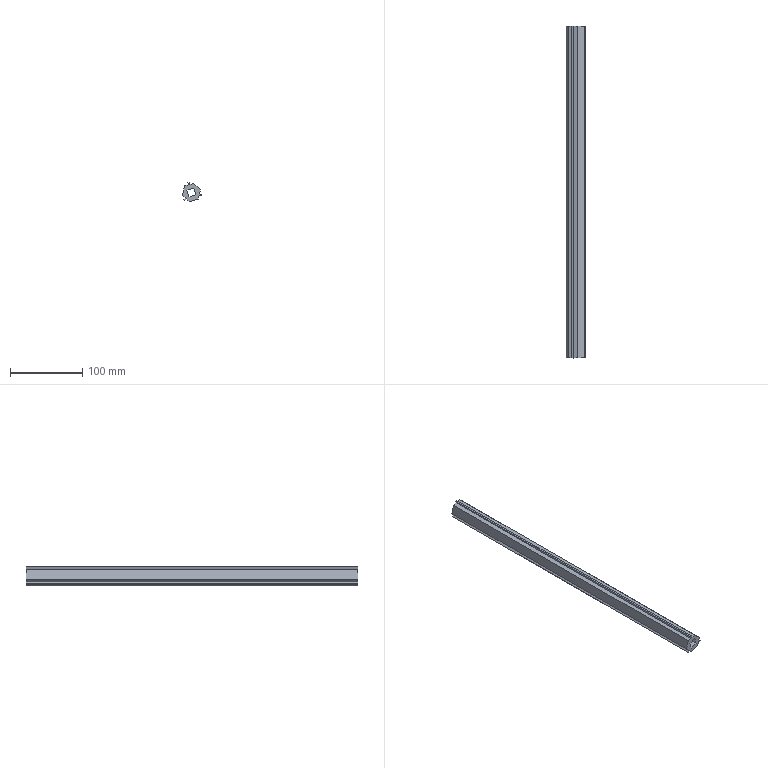Component | SolidWorks | Drive-1 | 1 solid | 24 faces | box 26.58 x 460 x 26.59 mm | volume 164254 mm3 | plane 24
STEP:
#1=CARTESIAN_POINT('',(-2.72,0.992,35.851));
#2=VERTEX_POINT('',#1);
#3=CARTESIAN_POINT('',(-2.928,0.992,35.792));
#4=VERTEX_POINT('',#3);
#5=CARTESIAN_POINT('',(-2.72,0.992,35.851));
#6=DIRECTION('',(-0.962,-0.,-0.273));
#7=VECTOR('',#6,39.37);
#8=LINE('',#5,#7);
#9=EDGE_CURVE('',#2,#4,#8,.T.);
#10=ORIENTED_EDGE('',*,*,#9,.T.);
#11=CARTESIAN_POINT('',(-3.053,0.992,35.296));
#12=VERTEX_POINT('',#11);
#13=CARTESIAN_POINT('',(-2.928,0.992,35.792));
#14=DIRECTION('',(-0.2446,0.,-0.9696));
#15=VECTOR('',#14,39.37);
#16=LINE('',#13,#15);
#17=EDGE_CURVE('',#4,#12,#16,.T.);
#18=ORIENTED_EDGE('',*,*,#17,.T.);
#19=CARTESIAN_POINT('',(-2.898,0.992,35.145));
#20=VERTEX_POINT('',#19);
#21=CARTESIAN_POINT('',(-3.053,0.992,35.296));
#22=DIRECTION('',(0.7175,0.,-0.6966));
#23=VECTOR('',#22,39.37);
#24=LINE('',#21,#23);
#25=EDGE_CURVE('',#12,#20,#24,.T.);
#26=ORIENTED_EDGE('',*,*,#25,.T.);
#27=CARTESIAN_POINT('',(-2.98,0.992,35.06));
#28=VERTEX_POINT('',#27);
#29=CARTESIAN_POINT('',(-2.898,0.992,35.145));
#30=DIRECTION('',(-0.6966,0.,-0.7175));
#31=VECTOR('',#30,39.37);
#32=LINE('',#29,#31);
#33=EDGE_CURVE('',#20,#28,#32,.T.);
#34=ORIENTED_EDGE('',*,*,#33,.T.);
#35=CARTESIAN_POINT('',(-2.924,0.992,35.005));
#36=VERTEX_POINT('',#35);
#37=CARTESIAN_POINT('',(-2.98,0.992,35.06));
#38=DIRECTION('',(0.7175,0.,-0.6966));
#39=VECTOR('',#38,39.37);
#40=LINE('',#37,#39);
#41=EDGE_CURVE('',#28,#36,#40,.T.);
#42=ORIENTED_EDGE('',*,*,#41,.T.);
#43=CARTESIAN_POINT('',(-2.841,0.992,35.09));
#44=VERTEX_POINT('',#43);
#45=CARTESIAN_POINT('',(-2.924,0.992,35.005));
#46=DIRECTION('',(0.6966,-0.,0.7175));
#47=VECTOR('',#46,39.37);
#48=LINE('',#45,#47);
#49=EDGE_CURVE('',#36,#44,#48,.T.);
#50=ORIENTED_EDGE('',*,*,#49,.T.);
#51=CARTESIAN_POINT('',(-2.686,0.992,34.939));
#52=VERTEX_POINT('',#51);
#53=CARTESIAN_POINT('',(-2.841,0.992,35.09));
#54=DIRECTION('',(0.7175,0.,-0.6966));
#55=VECTOR('',#54,39.37);
#56=LINE('',#53,#55);
#57=EDGE_CURVE('',#44,#52,#56,.T.);
#58=ORIENTED_EDGE('',*,*,#57,.T.);
#59=CARTESIAN_POINT('',(-2.194,0.992,35.079));
#60=VERTEX_POINT('',#59);
#61=CARTESIAN_POINT('',(-2.686,0.992,34.939));
#62=DIRECTION('',(0.962,0.,0.273));
#63=VECTOR('',#62,39.37);
#64=LINE('',#61,#63);
#65=EDGE_CURVE('',#52,#60,#64,.T.);
#66=ORIENTED_EDGE('',*,*,#65,.T.);
#67=CARTESIAN_POINT('',(-2.141,0.992,35.289));
#68=VERTEX_POINT('',#67);
#69=CARTESIAN_POINT('',(-2.194,0.992,35.079));
#70=DIRECTION('',(0.2446,-0.,0.9696));
#71=VECTOR('',#70,39.37);
#72=LINE('',#69,#71);
#73=EDGE_CURVE('',#60,#68,#72,.T.);
#74=ORIENTED_EDGE('',*,*,#73,.T.);
#75=CARTESIAN_POINT('',(-2.026,0.992,35.26));
#76=VERTEX_POINT('',#75);
#77=CARTESIAN_POINT('',(-2.026,0.992,35.26));
#78=DIRECTION('',(0.9696,0.,-0.2446));
#79=VECTOR('',#78,39.37);
#80=LINE('',#77,#79);
#81=EDGE_CURVE('',#68,#76,#80,.T.);
#82=ORIENTED_EDGE('',*,*,#81,.T.);
#83=CARTESIAN_POINT('',(-2.007,0.992,35.336));
#84=VERTEX_POINT('',#83);
#85=CARTESIAN_POINT('',(-2.007,0.992,35.336));
#86=DIRECTION('',(0.2446,-0.,0.9696));
#87=VECTOR('',#86,39.37);
#88=LINE('',#85,#87);
#89=EDGE_CURVE('',#76,#84,#88,.T.);
#90=ORIENTED_EDGE('',*,*,#89,.T.);
#91=CARTESIAN_POINT('',(-2.121,0.992,35.365));
#92=VERTEX_POINT('',#91);
#93=CARTESIAN_POINT('',(-2.121,0.992,35.365));
#94=DIRECTION('',(-0.9696,-0.,0.2446));
#95=VECTOR('',#94,39.37);
#96=LINE('',#93,#95);
#97=EDGE_CURVE('',#84,#92,#96,.T.);
#98=ORIENTED_EDGE('',*,*,#97,.T.);
#99=CARTESIAN_POINT('',(-2.068,0.992,35.575));
#100=VERTEX_POINT('',#99);
#101=CARTESIAN_POINT('',(-2.121,0.992,35.365));
#102=DIRECTION('',(0.2446,-0.,0.9696));
#103=VECTOR('',#102,39.37);
#104=LINE('',#101,#103);
#105=EDGE_CURVE('',#92,#100,#104,.T.);
#106=ORIENTED_EDGE('',*,*,#105,.T.);
#107=CARTESIAN_POINT('',(-2.436,0.992,35.932));
#108=VERTEX_POINT('',#107);
#109=CARTESIAN_POINT('',(-2.068,0.992,35.575));
#110=DIRECTION('',(-0.7175,-0.,0.6966));
#111=VECTOR('',#110,39.37);
#112=LINE('',#109,#111);
#113=EDGE_CURVE('',#100,#108,#112,.T.);
#114=ORIENTED_EDGE('',*,*,#113,.T.);
#115=CARTESIAN_POINT('',(-2.644,0.992,35.873));
#116=VERTEX_POINT('',#115);
#117=CARTESIAN_POINT('',(-2.436,0.992,35.932));
#118=DIRECTION('',(-0.962,-0.,-0.273));
#119=VECTOR('',#118,39.37);
#120=LINE('',#117,#119);
#121=EDGE_CURVE('',#108,#116,#120,.T.);
#122=ORIENTED_EDGE('',*,*,#121,.T.);
#123=CARTESIAN_POINT('',(-2.676,0.992,35.986));
#124=VERTEX_POINT('',#123);
#125=CARTESIAN_POINT('',(-2.676,0.992,35.986));
#126=DIRECTION('',(-0.273,-0.,0.962));
#127=VECTOR('',#126,39.37);
#128=LINE('',#125,#127);
#129=EDGE_CURVE('',#116,#124,#128,.T.);
#130=ORIENTED_EDGE('',*,*,#129,.T.);
#131=CARTESIAN_POINT('',(-2.752,0.992,35.965));
#132=VERTEX_POINT('',#131);
#133=CARTESIAN_POINT('',(-2.752,0.992,35.965));
#134=DIRECTION('',(-0.962,-0.,-0.273));
#135=VECTOR('',#134,39.37);
#136=LINE('',#133,#135);
#137=EDGE_CURVE('',#124,#132,#136,.T.);
#138=ORIENTED_EDGE('',*,*,#137,.T.);
#139=CARTESIAN_POINT('',(-2.72,0.992,35.851));
#140=DIRECTION('',(0.273,0.,-0.962));
#141=VECTOR('',#140,39.37);
#142=LINE('',#139,#141);
#143=EDGE_CURVE('',#132,#2,#142,.T.);
#144=ORIENTED_EDGE('',*,*,#143,.T.);
#145=EDGE_LOOP('',(#10,#18,#26,#34,#42,#50,#58,#66,#74,#82,#90,#98,#106,#114,#122,#130,#138,#144));
#146=FACE_OUTER_BOUND('',#145,.T.);
#147=CARTESIAN_POINT('',(-2.425,0.992,35.679));
#148=VERTEX_POINT('',#147);
#149=CARTESIAN_POINT('',(-2.804,0.992,35.571));
#150=VERTEX_POINT('',#149);
#151=CARTESIAN_POINT('',(-2.804,0.992,35.571));
#152=DIRECTION('',(-0.962,-0.,-0.273));
#153=VECTOR('',#152,39.37);
#154=LINE('',#151,#153);
#155=EDGE_CURVE('',#148,#150,#154,.T.);
#156=ORIENTED_EDGE('',*,*,#155,.F.);
#157=CARTESIAN_POINT('',(-2.318,0.992,35.3));
#158=VERTEX_POINT('',#157);
#159=CARTESIAN_POINT('',(-2.425,0.992,35.679));
#160=DIRECTION('',(-0.273,-0.,0.962));
#161=VECTOR('',#160,39.37);
#162=LINE('',#159,#161);
#163=EDGE_CURVE('',#158,#148,#162,.T.);
#164=ORIENTED_EDGE('',*,*,#163,.F.);
#165=CARTESIAN_POINT('',(-2.696,0.992,35.192));
#166=VERTEX_POINT('',#165);
#167=CARTESIAN_POINT('',(-2.696,0.992,35.192));
#168=DIRECTION('',(0.962,0.,0.273));
#169=VECTOR('',#168,39.37);
#170=LINE('',#167,#169);
#171=EDGE_CURVE('',#166,#158,#170,.T.);
#172=ORIENTED_EDGE('',*,*,#171,.F.);
#173=CARTESIAN_POINT('',(-2.804,0.992,35.571));
#174=DIRECTION('',(0.273,0.,-0.962));
#175=VECTOR('',#174,39.37);
#176=LINE('',#173,#175);
#177=EDGE_CURVE('',#150,#166,#176,.T.);
#178=ORIENTED_EDGE('',*,*,#177,.F.);
#179=EDGE_LOOP('',(#156,#164,#172,#178));
#180=FACE_BOUND('',#179,.T.);
#181=CARTESIAN_POINT('',(-2.561,0.992,35.436));
#182=DIRECTION('',(0.,-1.,-0.));
#183=DIRECTION('',(0.962,0.,0.273));
#184=AXIS2_PLACEMENT_3D('',#181,#182,#183);
#185=PLANE('',#184);
#186=ADVANCED_FACE('',(#146,#180),#185,.T.);
#187=CARTESIAN_POINT('',(-2.72,19.102,35.851));
#188=VERTEX_POINT('',#187);
#189=CARTESIAN_POINT('',(-2.928,19.102,35.792));
#190=VERTEX_POINT('',#189);
#191=CARTESIAN_POINT('',(-2.72,19.102,35.851));
#192=DIRECTION('',(-0.962,-0.,-0.273));
#193=VECTOR('',#192,39.37);
#194=LINE('',#191,#193);
#195=EDGE_CURVE('',#188,#190,#194,.T.);
#196=ORIENTED_EDGE('',*,*,#195,.F.);
#197=CARTESIAN_POINT('',(-2.752,19.102,35.965));
#198=VERTEX_POINT('',#197);
#199=CARTESIAN_POINT('',(-2.72,19.102,35.851));
#200=DIRECTION('',(0.273,0.,-0.962));
#201=VECTOR('',#200,39.37);
#202=LINE('',#199,#201);
#203=EDGE_CURVE('',#198,#188,#202,.T.);
#204=ORIENTED_EDGE('',*,*,#203,.F.);
#205=CARTESIAN_POINT('',(-2.676,19.102,35.986));
#206=VERTEX_POINT('',#205);
#207=CARTESIAN_POINT('',(-2.752,19.102,35.965));
#208=DIRECTION('',(-0.962,-0.,-0.273));
#209=VECTOR('',#208,39.37);
#210=LINE('',#207,#209);
#211=EDGE_CURVE('',#206,#198,#210,.T.);
#212=ORIENTED_EDGE('',*,*,#211,.F.);
#213=CARTESIAN_POINT('',(-2.644,19.102,35.873));
#214=VERTEX_POINT('',#213);
#215=CARTESIAN_POINT('',(-2.676,19.102,35.986));
#216=DIRECTION('',(-0.273,-0.,0.962));
#217=VECTOR('',#216,39.37);
#218=LINE('',#215,#217);
#219=EDGE_CURVE('',#214,#206,#218,.T.);
#220=ORIENTED_EDGE('',*,*,#219,.F.);
#221=CARTESIAN_POINT('',(-2.436,19.102,35.932));
#222=VERTEX_POINT('',#221);
#223=CARTESIAN_POINT('',(-2.436,19.102,35.932));
#224=DIRECTION('',(-0.962,-0.,-0.273));
#225=VECTOR('',#224,39.37);
#226=LINE('',#223,#225);
#227=EDGE_CURVE('',#222,#214,#226,.T.);
#228=ORIENTED_EDGE('',*,*,#227,.F.);
#229=CARTESIAN_POINT('',(-2.068,19.102,35.575));
#230=VERTEX_POINT('',#229);
#231=CARTESIAN_POINT('',(-2.068,19.102,35.575));
#232=DIRECTION('',(-0.7175,-0.,0.6966));
#233=VECTOR('',#232,39.37);
#234=LINE('',#231,#233);
#235=EDGE_CURVE('',#230,#222,#234,.T.);
#236=ORIENTED_EDGE('',*,*,#235,.F.);
#237=CARTESIAN_POINT('',(-2.121,19.102,35.365));
#238=VERTEX_POINT('',#237);
#239=CARTESIAN_POINT('',(-2.121,19.102,35.365));
#240=DIRECTION('',(0.2446,-0.,0.9696));
#241=VECTOR('',#240,39.37);
#242=LINE('',#239,#241);
#243=EDGE_CURVE('',#238,#230,#242,.T.);
#244=ORIENTED_EDGE('',*,*,#243,.F.);
#245=CARTESIAN_POINT('',(-2.007,19.102,35.336));
#246=VERTEX_POINT('',#245);
#247=CARTESIAN_POINT('',(-2.121,19.102,35.365));
#248=DIRECTION('',(-0.9696,-0.,0.2446));
#249=VECTOR('',#248,39.37);
#250=LINE('',#247,#249);
#251=EDGE_CURVE('',#246,#238,#250,.T.);
#252=ORIENTED_EDGE('',*,*,#251,.F.);
#253=CARTESIAN_POINT('',(-2.026,19.102,35.26));
#254=VERTEX_POINT('',#253);
#255=CARTESIAN_POINT('',(-2.007,19.102,35.336));
#256=DIRECTION('',(0.2446,-0.,0.9696));
#257=VECTOR('',#256,39.37);
#258=LINE('',#255,#257);
#259=EDGE_CURVE('',#254,#246,#258,.T.);
#260=ORIENTED_EDGE('',*,*,#259,.F.);
#261=CARTESIAN_POINT('',(-2.141,19.102,35.289));
#262=VERTEX_POINT('',#261);
#263=CARTESIAN_POINT('',(-2.026,19.102,35.26));
#264=DIRECTION('',(0.9696,0.,-0.2446));
#265=VECTOR('',#264,39.37);
#266=LINE('',#263,#265);
#267=EDGE_CURVE('',#262,#254,#266,.T.);
#268=ORIENTED_EDGE('',*,*,#267,.F.);
#269=CARTESIAN_POINT('',(-2.194,19.102,35.079));
#270=VERTEX_POINT('',#269);
#271=CARTESIAN_POINT('',(-2.194,19.102,35.079));
#272=DIRECTION('',(0.2446,-0.,0.9696));
#273=VECTOR('',#272,39.37);
#274=LINE('',#271,#273);
#275=EDGE_CURVE('',#270,#262,#274,.T.);
#276=ORIENTED_EDGE('',*,*,#275,.F.);
#277=CARTESIAN_POINT('',(-2.686,19.102,34.939));
#278=VERTEX_POINT('',#277);
#279=CARTESIAN_POINT('',(-2.686,19.102,34.939));
#280=DIRECTION('',(0.962,0.,0.273));
#281=VECTOR('',#280,39.37);
#282=LINE('',#279,#281);
#283=EDGE_CURVE('',#278,#270,#282,.T.);
#284=ORIENTED_EDGE('',*,*,#283,.F.);
#285=CARTESIAN_POINT('',(-2.841,19.102,35.09));
#286=VERTEX_POINT('',#285);
#287=CARTESIAN_POINT('',(-2.841,19.102,35.09));
#288=DIRECTION('',(0.7175,0.,-0.6966));
#289=VECTOR('',#288,39.37);
#290=LINE('',#287,#289);
#291=EDGE_CURVE('',#286,#278,#290,.T.);
#292=ORIENTED_EDGE('',*,*,#291,.F.);
#293=CARTESIAN_POINT('',(-2.924,19.102,35.005));
#294=VERTEX_POINT('',#293);
#295=CARTESIAN_POINT('',(-2.924,19.102,35.005));
#296=DIRECTION('',(0.6966,-0.,0.7175));
#297=VECTOR('',#296,39.37);
#298=LINE('',#295,#297);
#299=EDGE_CURVE('',#294,#286,#298,.T.);
#300=ORIENTED_EDGE('',*,*,#299,.F.);
#301=CARTESIAN_POINT('',(-2.98,19.102,35.06));
#302=VERTEX_POINT('',#301);
#303=CARTESIAN_POINT('',(-2.98,19.102,35.06));
#304=DIRECTION('',(0.7175,0.,-0.6966));
#305=VECTOR('',#304,39.37);
#306=LINE('',#303,#305);
#307=EDGE_CURVE('',#302,#294,#306,.T.);
#308=ORIENTED_EDGE('',*,*,#307,.F.);
#309=CARTESIAN_POINT('',(-2.898,19.102,35.145));
#310=VERTEX_POINT('',#309);
#311=CARTESIAN_POINT('',(-2.898,19.102,35.145));
#312=DIRECTION('',(-0.6966,0.,-0.7175));
#313=VECTOR('',#312,39.37);
#314=LINE('',#311,#313);
#315=EDGE_CURVE('',#310,#302,#314,.T.);
#316=ORIENTED_EDGE('',*,*,#315,.F.);
#317=CARTESIAN_POINT('',(-3.053,19.102,35.296));
#318=VERTEX_POINT('',#317);
#319=CARTESIAN_POINT('',(-3.053,19.102,35.296));
#320=DIRECTION('',(0.7175,0.,-0.6966));
#321=VECTOR('',#320,39.37);
#322=LINE('',#319,#321);
#323=EDGE_CURVE('',#318,#310,#322,.T.);
#324=ORIENTED_EDGE('',*,*,#323,.F.);
#325=CARTESIAN_POINT('',(-2.928,19.102,35.792));
#326=DIRECTION('',(-0.2446,0.,-0.9696));
#327=VECTOR('',#326,39.37);
#328=LINE('',#325,#327);
#329=EDGE_CURVE('',#190,#318,#328,.T.);
#330=ORIENTED_EDGE('',*,*,#329,.F.);
#331=EDGE_LOOP('',(#196,#204,#212,#220,#228,#236,#244,#252,#260,#268,#276,#284,#292,#300,#308,#316,#324,#330));
#332=FACE_OUTER_BOUND('',#331,.T.);
#333=CARTESIAN_POINT('',(-2.318,19.102,35.3));
#334=VERTEX_POINT('',#333);
#335=CARTESIAN_POINT('',(-2.425,19.102,35.679));
#336=VERTEX_POINT('',#335);
#337=CARTESIAN_POINT('',(-2.425,19.102,35.679));
#338=DIRECTION('',(-0.273,-0.,0.962));
#339=VECTOR('',#338,39.37);
#340=LINE('',#337,#339);
#341=EDGE_CURVE('',#334,#336,#340,.T.);
#342=ORIENTED_EDGE('',*,*,#341,.T.);
#343=CARTESIAN_POINT('',(-2.804,19.102,35.571));
#344=VERTEX_POINT('',#343);
#345=CARTESIAN_POINT('',(-2.804,19.102,35.571));
#346=DIRECTION('',(-0.962,-0.,-0.273));
#347=VECTOR('',#346,39.37);
#348=LINE('',#345,#347);
#349=EDGE_CURVE('',#336,#344,#348,.T.);
#350=ORIENTED_EDGE('',*,*,#349,.T.);
#351=CARTESIAN_POINT('',(-2.696,19.102,35.192));
#352=VERTEX_POINT('',#351);
#353=CARTESIAN_POINT('',(-2.804,19.102,35.571));
#354=DIRECTION('',(0.273,0.,-0.962));
#355=VECTOR('',#354,39.37);
#356=LINE('',#353,#355);
#357=EDGE_CURVE('',#344,#352,#356,.T.);
#358=ORIENTED_EDGE('',*,*,#357,.T.);
#359=CARTESIAN_POINT('',(-2.696,19.102,35.192));
#360=DIRECTION('',(0.962,0.,0.273));
#361=VECTOR('',#360,39.37);
#362=LINE('',#359,#361);
#363=EDGE_CURVE('',#352,#334,#362,.T.);
#364=ORIENTED_EDGE('',*,*,#363,.T.);
#365=EDGE_LOOP('',(#342,#350,#358,#364));
#366=FACE_BOUND('',#365,.T.);
#367=CARTESIAN_POINT('',(-2.561,19.102,35.436));
#368=DIRECTION('',(0.,-1.,-0.));
#369=DIRECTION('',(0.962,0.,0.273));
#370=AXIS2_PLACEMENT_3D('',#367,#368,#369);
#371=PLANE('',#370);
#372=ADVANCED_FACE('',(#332,#366),#371,.F.);
#373=ORIENTED_EDGE('',*,*,#195,.T.);
#374=CARTESIAN_POINT('',(-2.928,0.992,35.792));
#375=DIRECTION('',(-0.,1.,0.));
#376=VECTOR('',#375,39.37);
#377=LINE('',#374,#376);
#378=EDGE_CURVE('',#4,#190,#377,.T.);
#379=ORIENTED_EDGE('',*,*,#378,.F.);
#380=ORIENTED_EDGE('',*,*,#9,.F.);
#381=CARTESIAN_POINT('',(-2.72,0.992,35.851));
#382=DIRECTION('',(-0.,1.,0.));
#383=VECTOR('',#382,39.37);
#384=LINE('',#381,#383);
#385=EDGE_CURVE('',#2,#188,#384,.T.);
#386=ORIENTED_EDGE('',*,*,#385,.T.);
#387=EDGE_LOOP('',(#373,#379,#380,#386));
#388=FACE_OUTER_BOUND('',#387,.T.);
#389=CARTESIAN_POINT('',(-2.72,0.992,35.851));
#390=DIRECTION('',(0.273,0.,-0.962));
#391=DIRECTION('',(0.962,0.,0.273));
#392=AXIS2_PLACEMENT_3D('',#389,#390,#391);
#393=PLANE('',#392);
#394=ADVANCED_FACE('',(#388),#393,.F.);
#395=ORIENTED_EDGE('',*,*,#329,.T.);
#396=CARTESIAN_POINT('',(-3.053,0.992,35.296));
#397=DIRECTION('',(-0.,1.,0.));
#398=VECTOR('',#397,39.37);
#399=LINE('',#396,#398);
#400=EDGE_CURVE('',#12,#318,#399,.T.);
#401=ORIENTED_EDGE('',*,*,#400,.F.);
#402=ORIENTED_EDGE('',*,*,#17,.F.);
#403=ORIENTED_EDGE('',*,*,#378,.T.);
#404=EDGE_LOOP('',(#395,#401,#402,#403));
#405=FACE_OUTER_BOUND('',#404,.T.);
#406=CARTESIAN_POINT('',(-2.928,0.992,35.792));
#407=DIRECTION('',(0.9696,0.,-0.2446));
#408=DIRECTION('',(0.2446,-0.,0.9696));
#409=AXIS2_PLACEMENT_3D('',#406,#407,#408);
#410=PLANE('',#409);
#411=ADVANCED_FACE('',(#405),#410,.F.);
#412=ORIENTED_EDGE('',*,*,#323,.T.);
#413=CARTESIAN_POINT('',(-2.898,0.992,35.145));
#414=DIRECTION('',(-0.,1.,0.));
#415=VECTOR('',#414,39.37);
#416=LINE('',#413,#415);
#417=EDGE_CURVE('',#20,#310,#416,.T.);
#418=ORIENTED_EDGE('',*,*,#417,.F.);
#419=ORIENTED_EDGE('',*,*,#25,.F.);
#420=ORIENTED_EDGE('',*,*,#400,.T.);
#421=EDGE_LOOP('',(#412,#418,#419,#420));
#422=FACE_OUTER_BOUND('',#421,.T.);
#423=CARTESIAN_POINT('',(-3.053,0.992,35.296));
#424=DIRECTION('',(0.6966,-0.,0.7175));
#425=DIRECTION('',(-0.7175,-0.,0.6966));
#426=AXIS2_PLACEMENT_3D('',#423,#424,#425);
#427=PLANE('',#426);
#428=ADVANCED_FACE('',(#422),#427,.F.);
#429=ORIENTED_EDGE('',*,*,#315,.T.);
#430=CARTESIAN_POINT('',(-2.98,0.992,35.06));
#431=DIRECTION('',(-0.,1.,0.));
#432=VECTOR('',#431,39.37);
#433=LINE('',#430,#432);
#434=EDGE_CURVE('',#28,#302,#433,.T.);
#435=ORIENTED_EDGE('',*,*,#434,.F.);
#436=ORIENTED_EDGE('',*,*,#33,.F.);
#437=ORIENTED_EDGE('',*,*,#417,.T.);
#438=EDGE_LOOP('',(#429,#435,#436,#437));
#439=FACE_OUTER_BOUND('',#438,.T.);
#440=CARTESIAN_POINT('',(-2.898,0.992,35.145));
#441=DIRECTION('',(0.7175,0.,-0.6966));
#442=DIRECTION('',(0.6966,-0.,0.7175));
#443=AXIS2_PLACEMENT_3D('',#440,#441,#442);
#444=PLANE('',#443);
#445=ADVANCED_FACE('',(#439),#444,.F.);
#446=ORIENTED_EDGE('',*,*,#307,.T.);
#447=CARTESIAN_POINT('',(-2.924,0.992,35.005));
#448=DIRECTION('',(-0.,1.,0.));
#449=VECTOR('',#448,39.37);
#450=LINE('',#447,#449);
#451=EDGE_CURVE('',#36,#294,#450,.T.);
#452=ORIENTED_EDGE('',*,*,#451,.F.);
#453=ORIENTED_EDGE('',*,*,#41,.F.);
#454=ORIENTED_EDGE('',*,*,#434,.T.);
#455=EDGE_LOOP('',(#446,#452,#453,#454));
#456=FACE_OUTER_BOUND('',#455,.T.);
#457=CARTESIAN_POINT('',(-2.98,0.992,35.06));
#458=DIRECTION('',(0.6966,-0.,0.7175));
#459=DIRECTION('',(-0.7175,-0.,0.6966));
#460=AXIS2_PLACEMENT_3D('',#457,#458,#459);
#461=PLANE('',#460);
#462=ADVANCED_FACE('',(#456),#461,.F.);
#463=ORIENTED_EDGE('',*,*,#299,.T.);
#464=CARTESIAN_POINT('',(-2.841,0.992,35.09));
#465=DIRECTION('',(-0.,1.,0.));
#466=VECTOR('',#465,39.37);
#467=LINE('',#464,#466);
#468=EDGE_CURVE('',#44,#286,#467,.T.);
#469=ORIENTED_EDGE('',*,*,#468,.F.);
#470=ORIENTED_EDGE('',*,*,#49,.F.);
#471=ORIENTED_EDGE('',*,*,#451,.T.);
#472=EDGE_LOOP('',(#463,#469,#470,#471));
#473=FACE_OUTER_BOUND('',#472,.T.);
#474=CARTESIAN_POINT('',(-2.924,0.992,35.005));
#475=DIRECTION('',(-0.7175,-0.,0.6966));
#476=DIRECTION('',(-0.6966,0.,-0.7175));
#477=AXIS2_PLACEMENT_3D('',#474,#475,#476);
#478=PLANE('',#477);
#479=ADVANCED_FACE('',(#473),#478,.F.);
#480=ORIENTED_EDGE('',*,*,#291,.T.);
#481=CARTESIAN_POINT('',(-2.686,0.992,34.939));
#482=DIRECTION('',(-0.,1.,0.));
#483=VECTOR('',#482,39.37);
#484=LINE('',#481,#483);
#485=EDGE_CURVE('',#52,#278,#484,.T.);
#486=ORIENTED_EDGE('',*,*,#485,.F.);
#487=ORIENTED_EDGE('',*,*,#57,.F.);
#488=ORIENTED_EDGE('',*,*,#468,.T.);
#489=EDGE_LOOP('',(#480,#486,#487,#488));
#490=FACE_OUTER_BOUND('',#489,.T.);
#491=CARTESIAN_POINT('',(-2.841,0.992,35.09));
#492=DIRECTION('',(0.6966,-0.,0.7175));
#493=DIRECTION('',(-0.7175,-0.,0.6966));
#494=AXIS2_PLACEMENT_3D('',#491,#492,#493);
#495=PLANE('',#494);
#496=ADVANCED_FACE('',(#490),#495,.F.);
#497=ORIENTED_EDGE('',*,*,#283,.T.);
#498=CARTESIAN_POINT('',(-2.194,0.992,35.079));
#499=DIRECTION('',(-0.,1.,0.));
#500=VECTOR('',#499,39.37);
#501=LINE('',#498,#500);
#502=EDGE_CURVE('',#60,#270,#501,.T.);
#503=ORIENTED_EDGE('',*,*,#502,.F.);
#504=ORIENTED_EDGE('',*,*,#65,.F.);
#505=ORIENTED_EDGE('',*,*,#485,.T.);
#506=EDGE_LOOP('',(#497,#503,#504,#505));
#507=FACE_OUTER_BOUND('',#506,.T.);
#508=CARTESIAN_POINT('',(-2.686,0.992,34.939));
#509=DIRECTION('',(-0.273,-0.,0.962));
#510=DIRECTION('',(-0.962,-0.,-0.273));
#511=AXIS2_PLACEMENT_3D('',#508,#509,#510);
#512=PLANE('',#511);
#513=ADVANCED_FACE('',(#507),#512,.F.);
#514=ORIENTED_EDGE('',*,*,#275,.T.);
#515=CARTESIAN_POINT('',(-2.141,0.992,35.289));
#516=DIRECTION('',(-0.,1.,0.));
#517=VECTOR('',#516,39.37);
#518=LINE('',#515,#517);
#519=EDGE_CURVE('',#68,#262,#518,.T.);
#520=ORIENTED_EDGE('',*,*,#519,.F.);
#521=ORIENTED_EDGE('',*,*,#73,.F.);
#522=ORIENTED_EDGE('',*,*,#502,.T.);
#523=EDGE_LOOP('',(#514,#520,#521,#522));
#524=FACE_OUTER_BOUND('',#523,.T.);
#525=CARTESIAN_POINT('',(-2.194,0.992,35.079));
#526=DIRECTION('',(-0.9696,-0.,0.2446));
#527=DIRECTION('',(-0.2446,0.,-0.9696));
#528=AXIS2_PLACEMENT_3D('',#525,#526,#527);
#529=PLANE('',#528);
#530=ADVANCED_FACE('',(#524),#529,.F.);
#531=ORIENTED_EDGE('',*,*,#267,.T.);
#532=CARTESIAN_POINT('',(-2.026,0.992,35.26));
#533=DIRECTION('',(-0.,1.,0.));
#534=VECTOR('',#533,39.37);
#535=LINE('',#532,#534);
#536=EDGE_CURVE('',#76,#254,#535,.T.);
#537=ORIENTED_EDGE('',*,*,#536,.F.);
#538=ORIENTED_EDGE('',*,*,#81,.F.);
#539=ORIENTED_EDGE('',*,*,#519,.T.);
#540=EDGE_LOOP('',(#531,#537,#538,#539));
#541=FACE_OUTER_BOUND('',#540,.T.);
#542=CARTESIAN_POINT('',(-2.026,0.992,35.26));
#543=DIRECTION('',(0.2446,-0.,0.9696));
#544=DIRECTION('',(-0.9696,-0.,0.2446));
#545=AXIS2_PLACEMENT_3D('',#542,#543,#544);
#546=PLANE('',#545);
#547=ADVANCED_FACE('',(#541),#546,.F.);
#548=ORIENTED_EDGE('',*,*,#259,.T.);
#549=CARTESIAN_POINT('',(-2.007,0.992,35.336));
#550=DIRECTION('',(-0.,1.,0.));
#551=VECTOR('',#550,39.37);
#552=LINE('',#549,#551);
#553=EDGE_CURVE('',#84,#246,#552,.T.);
#554=ORIENTED_EDGE('',*,*,#553,.F.);
#555=ORIENTED_EDGE('',*,*,#89,.F.);
#556=ORIENTED_EDGE('',*,*,#536,.T.);
#557=EDGE_LOOP('',(#548,#554,#555,#556));
#558=FACE_OUTER_BOUND('',#557,.T.);
#559=CARTESIAN_POINT('',(-2.007,0.992,35.336));
#560=DIRECTION('',(-0.9696,-0.,0.2446));
#561=DIRECTION('',(-0.2446,0.,-0.9696));
#562=AXIS2_PLACEMENT_3D('',#559,#560,#561);
#563=PLANE('',#562);
#564=ADVANCED_FACE('',(#558),#563,.F.);
#565=ORIENTED_EDGE('',*,*,#251,.T.);
#566=CARTESIAN_POINT('',(-2.121,0.992,35.365));
#567=DIRECTION('',(-0.,1.,0.));
#568=VECTOR('',#567,39.37);
#569=LINE('',#566,#568);
#570=EDGE_CURVE('',#92,#238,#569,.T.);
#571=ORIENTED_EDGE('',*,*,#570,.F.);
#572=ORIENTED_EDGE('',*,*,#97,.F.);
#573=ORIENTED_EDGE('',*,*,#553,.T.);
#574=EDGE_LOOP('',(#565,#571,#572,#573));
#575=FACE_OUTER_BOUND('',#574,.T.);
#576=CARTESIAN_POINT('',(-2.121,0.992,35.365));
#577=DIRECTION('',(-0.2446,0.,-0.9696));
#578=DIRECTION('',(0.9696,0.,-0.2446));
#579=AXIS2_PLACEMENT_3D('',#576,#577,#578);
#580=PLANE('',#579);
#581=ADVANCED_FACE('',(#575),#580,.F.);
#582=ORIENTED_EDGE('',*,*,#243,.T.);
#583=CARTESIAN_POINT('',(-2.068,0.992,35.575));
#584=DIRECTION('',(-0.,1.,0.));
#585=VECTOR('',#584,39.37);
#586=LINE('',#583,#585);
#587=EDGE_CURVE('',#100,#230,#586,.T.);
#588=ORIENTED_EDGE('',*,*,#587,.F.);
#589=ORIENTED_EDGE('',*,*,#105,.F.);
#590=ORIENTED_EDGE('',*,*,#570,.T.);
#591=EDGE_LOOP('',(#582,#588,#589,#590));
#592=FACE_OUTER_BOUND('',#591,.T.);
#593=CARTESIAN_POINT('',(-2.121,0.992,35.365));
#594=DIRECTION('',(-0.9696,-0.,0.2446));
#595=DIRECTION('',(-0.2446,0.,-0.9696));
#596=AXIS2_PLACEMENT_3D('',#593,#594,#595);
#597=PLANE('',#596);
#598=ADVANCED_FACE('',(#592),#597,.F.);
#599=ORIENTED_EDGE('',*,*,#235,.T.);
#600=CARTESIAN_POINT('',(-2.436,0.992,35.932));
#601=DIRECTION('',(-0.,1.,0.));
#602=VECTOR('',#601,39.37);
#603=LINE('',#600,#602);
#604=EDGE_CURVE('',#108,#222,#603,.T.);
#605=ORIENTED_EDGE('',*,*,#604,.F.);
#606=ORIENTED_EDGE('',*,*,#113,.F.);
#607=ORIENTED_EDGE('',*,*,#587,.T.);
#608=EDGE_LOOP('',(#599,#605,#606,#607));
#609=FACE_OUTER_BOUND('',#608,.T.);
#610=CARTESIAN_POINT('',(-2.068,0.992,35.575));
#611=DIRECTION('',(-0.6966,0.,-0.7175));
#612=DIRECTION('',(0.7175,0.,-0.6966));
#613=AXIS2_PLACEMENT_3D('',#610,#611,#612);
#614=PLANE('',#613);
#615=ADVANCED_FACE('',(#609),#614,.F.);
#616=ORIENTED_EDGE('',*,*,#227,.T.);
#617=CARTESIAN_POINT('',(-2.644,0.992,35.873));
#618=DIRECTION('',(-0.,1.,0.));
#619=VECTOR('',#618,39.37);
#620=LINE('',#617,#619);
#621=EDGE_CURVE('',#116,#214,#620,.T.);
#622=ORIENTED_EDGE('',*,*,#621,.F.);
#623=ORIENTED_EDGE('',*,*,#121,.F.);
#624=ORIENTED_EDGE('',*,*,#604,.T.);
#625=EDGE_LOOP('',(#616,#622,#623,#624));
#626=FACE_OUTER_BOUND('',#625,.T.);
#627=CARTESIAN_POINT('',(-2.436,0.992,35.932));
#628=DIRECTION('',(0.273,0.,-0.962));
#629=DIRECTION('',(0.962,0.,0.273));
#630=AXIS2_PLACEMENT_3D('',#627,#628,#629);
#631=PLANE('',#630);
#632=ADVANCED_FACE('',(#626),#631,.F.);
#633=ORIENTED_EDGE('',*,*,#219,.T.);
#634=CARTESIAN_POINT('',(-2.676,0.992,35.986));
#635=DIRECTION('',(-0.,1.,0.));
#636=VECTOR('',#635,39.37);
#637=LINE('',#634,#636);
#638=EDGE_CURVE('',#124,#206,#637,.T.);
#639=ORIENTED_EDGE('',*,*,#638,.F.);
#640=ORIENTED_EDGE('',*,*,#129,.F.);
#641=ORIENTED_EDGE('',*,*,#621,.T.);
#642=EDGE_LOOP('',(#633,#639,#640,#641));
#643=FACE_OUTER_BOUND('',#642,.T.);
#644=CARTESIAN_POINT('',(-2.676,0.992,35.986));
#645=DIRECTION('',(-0.962,-0.,-0.273));
#646=DIRECTION('',(0.,-1.,-0.));
#647=AXIS2_PLACEMENT_3D('',#644,#645,#646);
#648=PLANE('',#647);
#649=ADVANCED_FACE('',(#643),#648,.F.);
#650=ORIENTED_EDGE('',*,*,#211,.T.);
#651=CARTESIAN_POINT('',(-2.752,0.992,35.965));
#652=DIRECTION('',(-0.,1.,0.));
#653=VECTOR('',#652,39.37);
#654=LINE('',#651,#653);
#655=EDGE_CURVE('',#132,#198,#654,.T.);
#656=ORIENTED_EDGE('',*,*,#655,.F.);
#657=ORIENTED_EDGE('',*,*,#137,.F.);
#658=ORIENTED_EDGE('',*,*,#638,.T.);
#659=EDGE_LOOP('',(#650,#656,#657,#658));
#660=FACE_OUTER_BOUND('',#659,.T.);
#661=CARTESIAN_POINT('',(-2.752,0.992,35.965));
#662=DIRECTION('',(0.273,0.,-0.962));
#663=DIRECTION('',(-0.,1.,0.));
#664=AXIS2_PLACEMENT_3D('',#661,#662,#663);
#665=PLANE('',#664);
#666=ADVANCED_FACE('',(#660),#665,.F.);
#667=ORIENTED_EDGE('',*,*,#203,.T.);
#668=ORIENTED_EDGE('',*,*,#385,.F.);
#669=ORIENTED_EDGE('',*,*,#143,.F.);
#670=ORIENTED_EDGE('',*,*,#655,.T.);
#671=EDGE_LOOP('',(#667,#668,#669,#670));
#672=FACE_OUTER_BOUND('',#671,.T.);
#673=CARTESIAN_POINT('',(-2.72,0.992,35.851));
#674=DIRECTION('',(0.962,0.,0.273));
#675=DIRECTION('',(-0.,1.,0.));
#676=AXIS2_PLACEMENT_3D('',#673,#674,#675);
#677=PLANE('',#676);
#678=ADVANCED_FACE('',(#672),#677,.F.);
#679=ORIENTED_EDGE('',*,*,#341,.F.);
#680=CARTESIAN_POINT('',(-2.318,0.992,35.3));
#681=DIRECTION('',(-0.,1.,0.));
#682=VECTOR('',#681,39.37);
#683=LINE('',#680,#682);
#684=EDGE_CURVE('',#158,#334,#683,.T.);
#685=ORIENTED_EDGE('',*,*,#684,.F.);
#686=ORIENTED_EDGE('',*,*,#163,.T.);
#687=CARTESIAN_POINT('',(-2.425,0.992,35.679));
#688=DIRECTION('',(-0.,1.,0.));
#689=VECTOR('',#688,39.37);
#690=LINE('',#687,#689);
#691=EDGE_CURVE('',#148,#336,#690,.T.);
#692=ORIENTED_EDGE('',*,*,#691,.T.);
#693=EDGE_LOOP('',(#679,#685,#686,#692));
#694=FACE_OUTER_BOUND('',#693,.T.);
#695=CARTESIAN_POINT('',(-2.425,0.992,35.679));
#696=DIRECTION('',(-0.962,-0.,-0.273));
#697=DIRECTION('',(0.273,0.,-0.962));
#698=AXIS2_PLACEMENT_3D('',#695,#696,#697);
#699=PLANE('',#698);
#700=ADVANCED_FACE('',(#694),#699,.T.);
#701=ORIENTED_EDGE('',*,*,#349,.F.);
#702=ORIENTED_EDGE('',*,*,#691,.F.);
#703=ORIENTED_EDGE('',*,*,#155,.T.);
#704=CARTESIAN_POINT('',(-2.804,0.992,35.571));
#705=DIRECTION('',(-0.,1.,0.));
#706=VECTOR('',#705,39.37);
#707=LINE('',#704,#706);
#708=EDGE_CURVE('',#150,#344,#707,.T.);
#709=ORIENTED_EDGE('',*,*,#708,.T.);
#710=EDGE_LOOP('',(#701,#702,#703,#709));
#711=FACE_OUTER_BOUND('',#710,.T.);
#712=CARTESIAN_POINT('',(-2.804,0.992,35.571));
#713=DIRECTION('',(0.273,0.,-0.962));
#714=DIRECTION('',(-0.,1.,0.));
#715=AXIS2_PLACEMENT_3D('',#712,#713,#714);
#716=PLANE('',#715);
#717=ADVANCED_FACE('',(#711),#716,.T.);
#718=ORIENTED_EDGE('',*,*,#357,.F.);
#719=ORIENTED_EDGE('',*,*,#708,.F.);
#720=ORIENTED_EDGE('',*,*,#177,.T.);
#721=CARTESIAN_POINT('',(-2.696,0.992,35.192));
#722=DIRECTION('',(-0.,1.,0.));
#723=VECTOR('',#722,39.37);
#724=LINE('',#721,#723);
#725=EDGE_CURVE('',#166,#352,#724,.T.);
#726=ORIENTED_EDGE('',*,*,#725,.T.);
#727=EDGE_LOOP('',(#718,#719,#720,#726));
#728=FACE_OUTER_BOUND('',#727,.T.);
#729=CARTESIAN_POINT('',(-2.804,0.992,35.571));
#730=DIRECTION('',(0.962,0.,0.273));
#731=DIRECTION('',(-0.273,-0.,0.962));
#732=AXIS2_PLACEMENT_3D('',#729,#730,#731);
#733=PLANE('',#732);
#734=ADVANCED_FACE('',(#728),#733,.T.);
#735=ORIENTED_EDGE('',*,*,#363,.F.);
#736=ORIENTED_EDGE('',*,*,#725,.F.);
#737=ORIENTED_EDGE('',*,*,#171,.T.);
#738=ORIENTED_EDGE('',*,*,#684,.T.);
#739=EDGE_LOOP('',(#735,#736,#737,#738));
#740=FACE_OUTER_BOUND('',#739,.T.);
#741=CARTESIAN_POINT('',(-2.696,0.992,35.192));
#742=DIRECTION('',(-0.273,-0.,0.962));
#743=DIRECTION('',(0.,-1.,-0.));
#744=AXIS2_PLACEMENT_3D('',#741,#742,#743);
#745=PLANE('',#744);
#746=ADVANCED_FACE('',(#740),#745,.T.);
#747=CLOSED_SHELL('',(#186,#372,#394,#411,#428,#445,#462,#479,#496,#513,#530,#547,#564,#581,#598,#615,#632,#649,#666,#678,#700,#717,#734,#746));
#748=MANIFOLD_SOLID_BREP('',#747);
#749=CARTESIAN_POINT('',(0.,0.,0.));
#750=DIRECTION('',(0.,0.,1.));
#751=DIRECTION('',(1.,0.,0.));
#752=AXIS2_PLACEMENT_3D('',#749,#750,#751);
#753=(LENGTH_UNIT()NAMED_UNIT(*)SI_UNIT($,.METRE.));
#754=LENGTH_MEASURE_WITH_UNIT(LENGTH_MEASURE(0.0254),#753);
#755=DIMENSIONAL_EXPONENTS(1.,0.,0.,0.,0.,0.,0.);
#756=(CONVERSION_BASED_UNIT('',#754)LENGTH_UNIT()NAMED_UNIT(#755));
#757=UNCERTAINTY_MEASURE_WITH_UNIT(LENGTH_MEASURE(0.00001),#756,'','');
#758=(NAMED_UNIT(*)PLANE_ANGLE_UNIT()SI_UNIT($,.RADIAN.));
#759=(NAMED_UNIT(*)SI_UNIT($,.STERADIAN.)SOLID_ANGLE_UNIT());
#760=(GEOMETRIC_REPRESENTATION_CONTEXT(3)GLOBAL_UNCERTAINTY_ASSIGNED_CONTEXT((#757))GLOBAL_UNIT_ASSIGNED_CONTEXT((#756,#758,#759))REPRESENTATION_CONTEXT('',''));
#761=ADVANCED_BREP_SHAPE_REPRESENTATION('',(#748,#752),#760);
#762=COLOUR_RGB('',0.7922,0.8196,0.9333);
#763=FILL_AREA_STYLE_COLOUR('',#762);
#764=FILL_AREA_STYLE('',(#763));
#765=SURFACE_STYLE_FILL_AREA(#764);
#766=SURFACE_SIDE_STYLE('',(#765));
#767=SURFACE_STYLE_USAGE(.BOTH.,#766);
#768=PRESENTATION_STYLE_ASSIGNMENT((#767));
#769=STYLED_ITEM('',(#768),#748);
#770=(LENGTH_UNIT()NAMED_UNIT(*)SI_UNIT($,.METRE.));
#771=LENGTH_MEASURE_WITH_UNIT(LENGTH_MEASURE(0.0254),#770);
#772=DIMENSIONAL_EXPONENTS(1.,0.,0.,0.,0.,0.,0.);
#773=(CONVERSION_BASED_UNIT('',#771)LENGTH_UNIT()NAMED_UNIT(#772));
#774=UNCERTAINTY_MEASURE_WITH_UNIT(LENGTH_MEASURE(0.00001),#773,'','');
#775=(NAMED_UNIT(*)PLANE_ANGLE_UNIT()SI_UNIT($,.RADIAN.));
#776=(NAMED_UNIT(*)SI_UNIT($,.STERADIAN.)SOLID_ANGLE_UNIT());
#777=(GEOMETRIC_REPRESENTATION_CONTEXT(3)GLOBAL_UNCERTAINTY_ASSIGNED_CONTEXT((#774))GLOBAL_UNIT_ASSIGNED_CONTEXT((#773,#775,#776))REPRESENTATION_CONTEXT('',''));
#778=MECHANICAL_DESIGN_GEOMETRIC_PRESENTATION_REPRESENTATION('',(#769),#777);
#779=PRESENTATION_LAYER_ASSIGNMENT('','',(#769));